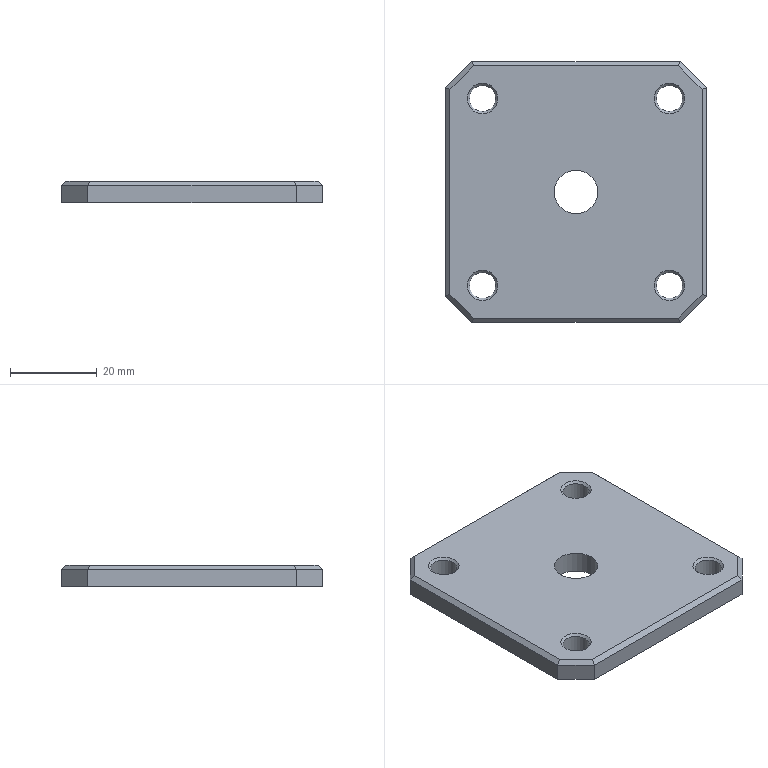Component | NX | CYLINDER_COVER | 1 solid | 31 faces | volume 16550 mm3 | plane 18 | cone 8 | cylinder 5 | commonest cylinder face diameters 6 x4 10 x1